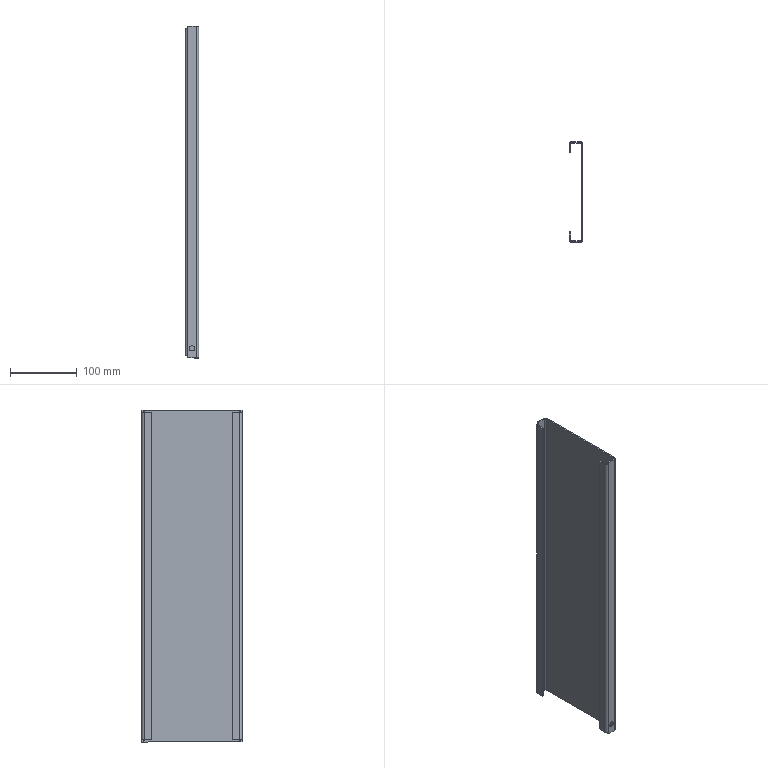Component | SolidWorks | BoxWelding-1_AuxiliaryPanel2-1 | 1 solid | 44 faces | volume 204698 mm3 | plane 34 | cylinder 10 | commonest cylinder face diameters 8 x6 4 x4